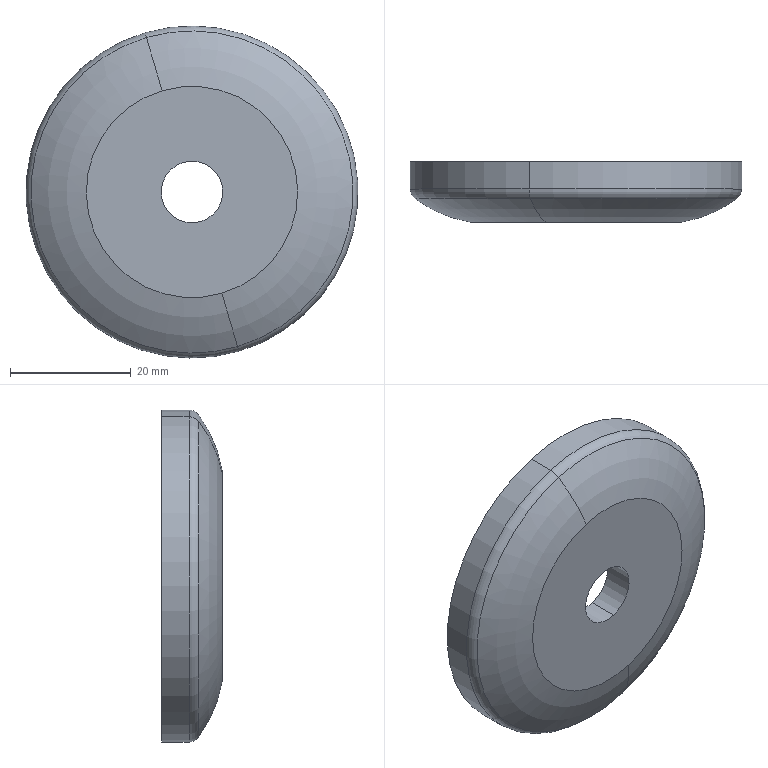Component | SolidWorks | Blade cover-1 | 1 solid | 19 faces | box 55 x 10 x 55 mm | volume 12758 mm3 | cylinder 10 | plane 5 | torus 4 | commonest cylinder face diameters 55 x2 10.2 x2 30 x2 36 x2 49 x2
build123d program:
from build123d import *

# Parameters (mm, degrees)
CONG_1_R = 2


with BuildPart() as part:
    # Esquisse1 → R_volution1 (revolve)
    with BuildSketch(Plane.XY, mode=Mode.PRIVATE) as r_volution1_sk:
        with BuildLine():
            Line((27.5, 0), (27.5, 5.5))
            ThreePointArc((27.5, 5.5), (22.785, 8.383), (17.5, 10))
            Line((17.5, 10), (5.1, 10))
            Line((5.1, 10), (5.1, 5))
            Line((5.1, 5), (15, 5))
            Line((15, 5), (15, 0))
            Line((15, 0), (18, 0))
            Line((18, 0), (18, 5))
            Line((18, 5), (24.5, 5))
            Line((24.5, 5), (24.5, 0))
            Line((24.5, 0), (27.5, 0))
        make_face()
    revolve(r_volution1_sk.sketch.rotate(Axis((0, 0, 0), (0, 1, 0)), 90), axis=Axis((0, 0, 0), (0, 1, 0)))

    # Cong_1
    cong_1_edges = [part.edges().sort_by_distance(p)[0] for p in [
        (0, 5.5, 27.5),
    ]]
    fillet(cong_1_edges, radius=CONG_1_R)


solid = part.part

# Placed as in the assembly
solid = solid.moved(Location((-11.038, -39.3, -47.854), (180, 0, 0)))
STEP:
#1=COLOUR_RGB('',0.7922,0.8196,0.9333);
#2=FILL_AREA_STYLE_COLOUR('',#1);
#3=FILL_AREA_STYLE('',(#2));
#4=SURFACE_STYLE_FILL_AREA(#3);
#5=SURFACE_SIDE_STYLE('',(#4));
#6=SURFACE_STYLE_USAGE(.BOTH.,#5);
#7=PRESENTATION_STYLE_ASSIGNMENT((#6));
#8=CARTESIAN_POINT('',(-0.7406,-1.725,-0.8455));
#9=VERTEX_POINT('',#8);
#10=CARTESIAN_POINT('',(-0.1285,-1.725,-2.923));
#11=VERTEX_POINT('',#10);
#12=CARTESIAN_POINT('',(-0.4346,-1.725,-1.884));
#13=DIRECTION('',(0.,1.,-0.));
#14=DIRECTION('',(0.2827,-0.,-0.9592));
#15=AXIS2_PLACEMENT_3D('',#12,#13,#14);
#16=CIRCLE('',#15,1.083);
#17=EDGE_CURVE('',#9,#11,#16,.T.);
#18=ORIENTED_EDGE('',*,*,#17,.F.);
#19=CARTESIAN_POINT('',(-0.7314,-1.789,-0.8767));
#20=VERTEX_POINT('',#19);
#21=CARTESIAN_POINT('',(-0.7184,-1.725,-0.921));
#22=DIRECTION('',(0.9592,-0.,0.2827));
#23=DIRECTION('',(0.2827,0.,-0.9592));
#24=AXIS2_PLACEMENT_3D('',#21,#22,#23);
#25=CIRCLE('',#24,0.07874);
#26=EDGE_CURVE('',#9,#20,#25,.T.);
#27=ORIENTED_EDGE('',*,*,#26,.T.);
#28=CARTESIAN_POINT('',(-0.1377,-1.789,-2.891));
#29=VERTEX_POINT('',#28);
#30=CARTESIAN_POINT('',(-0.4346,-1.789,-1.884));
#31=DIRECTION('',(-0.,-1.,0.));
#32=DIRECTION('',(-0.2827,0.,0.9592));
#33=AXIS2_PLACEMENT_3D('',#30,#31,#32);
#34=CIRCLE('',#33,1.05);
#35=EDGE_CURVE('',#29,#20,#34,.T.);
#36=ORIENTED_EDGE('',*,*,#35,.F.);
#37=CARTESIAN_POINT('',(-0.1508,-1.725,-2.847));
#38=DIRECTION('',(-0.9592,0.,-0.2827));
#39=DIRECTION('',(-0.2827,0.,0.9592));
#40=AXIS2_PLACEMENT_3D('',#37,#38,#39);
#41=CIRCLE('',#40,0.07874);
#42=EDGE_CURVE('',#11,#29,#41,.T.);
#43=ORIENTED_EDGE('',*,*,#42,.F.);
#44=EDGE_LOOP('',(#18,#27,#36,#43));
#45=FACE_OUTER_BOUND('',#44,.T.);
#46=CARTESIAN_POINT('',(-0.4346,-1.725,-1.884));
#47=DIRECTION('',(-0.,-1.,0.));
#48=DIRECTION('',(0.2827,-0.,-0.9592));
#49=AXIS2_PLACEMENT_3D('',#46,#47,#48);
#50=TOROIDAL_SURFACE('',#49,1.004,0.07874);
#51=ADVANCED_FACE('',(#45),#50,.T.);
#52=ORIENTED_EDGE('',*,*,#17,.T.);
#53=CARTESIAN_POINT('',(-0.1285,-1.547,-2.923));
#54=VERTEX_POINT('',#53);
#55=CARTESIAN_POINT('',(-0.1285,-1.547,-2.923));
#56=DIRECTION('',(0.,1.,-0.));
#57=VECTOR('',#56,39.37);
#58=LINE('',#55,#57);
#59=EDGE_CURVE('',#11,#54,#58,.T.);
#60=ORIENTED_EDGE('',*,*,#59,.T.);
#61=CARTESIAN_POINT('',(-0.7406,-1.547,-0.8455));
#62=VERTEX_POINT('',#61);
#63=CARTESIAN_POINT('',(-0.4346,-1.547,-1.884));
#64=DIRECTION('',(0.,1.,-0.));
#65=DIRECTION('',(-0.2827,0.,0.9592));
#66=AXIS2_PLACEMENT_3D('',#63,#64,#65);
#67=CIRCLE('',#66,1.083);
#68=EDGE_CURVE('',#62,#54,#67,.T.);
#69=ORIENTED_EDGE('',*,*,#68,.F.);
#70=CARTESIAN_POINT('',(-0.7406,-1.547,-0.8455));
#71=DIRECTION('',(0.,1.,-0.));
#72=VECTOR('',#71,39.37);
#73=LINE('',#70,#72);
#74=EDGE_CURVE('',#9,#62,#73,.T.);
#75=ORIENTED_EDGE('',*,*,#74,.F.);
#76=EDGE_LOOP('',(#52,#60,#69,#75));
#77=FACE_OUTER_BOUND('',#76,.T.);
#78=CARTESIAN_POINT('',(-0.4346,-1.547,-1.884));
#79=DIRECTION('',(0.,1.,-0.));
#80=DIRECTION('',(-0.2827,0.,0.9592));
#81=AXIS2_PLACEMENT_3D('',#78,#79,#80);
#82=CYLINDRICAL_SURFACE('',#81,1.083);
#83=ADVANCED_FACE('',(#77),#82,.T.);
#84=CARTESIAN_POINT('',(-0.6293,-1.941,-1.223));
#85=VERTEX_POINT('',#84);
#86=CARTESIAN_POINT('',(-0.2398,-1.941,-2.545));
#87=VERTEX_POINT('',#86);
#88=CARTESIAN_POINT('',(-0.4346,-1.941,-1.884));
#89=DIRECTION('',(0.,1.,-0.));
#90=DIRECTION('',(-0.2827,0.,0.9592));
#91=AXIS2_PLACEMENT_3D('',#88,#89,#90);
#92=CIRCLE('',#91,0.689);
#93=EDGE_CURVE('',#85,#87,#92,.T.);
#94=ORIENTED_EDGE('',*,*,#93,.T.);
#95=CARTESIAN_POINT('',(-0.2815,-1.087,-2.404));
#96=DIRECTION('',(0.9592,-0.,0.2827));
#97=DIRECTION('',(0.2827,0.,-0.9592));
#98=AXIS2_PLACEMENT_3D('',#95,#96,#97);
#99=CIRCLE('',#98,0.8661);
#100=EDGE_CURVE('',#87,#29,#99,.T.);
#101=ORIENTED_EDGE('',*,*,#100,.T.);
#102=ORIENTED_EDGE('',*,*,#35,.T.);
#103=CARTESIAN_POINT('',(-0.5877,-1.087,-1.365));
#104=DIRECTION('',(-0.9592,0.,-0.2827));
#105=DIRECTION('',(-0.2827,0.,0.9592));
#106=AXIS2_PLACEMENT_3D('',#103,#104,#105);
#107=CIRCLE('',#106,0.8661);
#108=EDGE_CURVE('',#85,#20,#107,.T.);
#109=ORIENTED_EDGE('',*,*,#108,.F.);
#110=EDGE_LOOP('',(#94,#101,#102,#109));
#111=FACE_OUTER_BOUND('',#110,.T.);
#112=CARTESIAN_POINT('',(-0.4346,-1.087,-1.884));
#113=DIRECTION('',(0.,1.,-0.));
#114=DIRECTION('',(-0.2827,0.,0.9592));
#115=AXIS2_PLACEMENT_3D('',#112,#113,#114);
#116=TOROIDAL_SURFACE('',#115,0.5416,0.8661);
#117=ADVANCED_FACE('',(#111),#116,.T.);
#118=CARTESIAN_POINT('',(-0.3778,-1.941,-2.077));
#119=VERTEX_POINT('',#118);
#120=CARTESIAN_POINT('',(-0.4913,-1.941,-1.691));
#121=VERTEX_POINT('',#120);
#122=CARTESIAN_POINT('',(-0.4346,-1.941,-1.884));
#123=DIRECTION('',(0.,1.,-0.));
#124=DIRECTION('',(-0.2827,0.,0.9592));
#125=AXIS2_PLACEMENT_3D('',#122,#123,#124);
#126=CIRCLE('',#125,0.2008);
#127=EDGE_CURVE('',#119,#121,#126,.T.);
#128=ORIENTED_EDGE('',*,*,#127,.F.);
#129=CARTESIAN_POINT('',(-0.3778,-1.744,-2.077));
#130=VERTEX_POINT('',#129);
#131=CARTESIAN_POINT('',(-0.3778,-1.547,-2.077));
#132=DIRECTION('',(0.,1.,-0.));
#133=VECTOR('',#132,39.37);
#134=LINE('',#131,#133);
#135=EDGE_CURVE('',#119,#130,#134,.T.);
#136=ORIENTED_EDGE('',*,*,#135,.T.);
#137=CARTESIAN_POINT('',(-0.4913,-1.744,-1.691));
#138=VERTEX_POINT('',#137);
#139=CARTESIAN_POINT('',(-0.4346,-1.744,-1.884));
#140=DIRECTION('',(0.,1.,-0.));
#141=DIRECTION('',(-0.2827,0.,0.9592));
#142=AXIS2_PLACEMENT_3D('',#139,#140,#141);
#143=CIRCLE('',#142,0.2008);
#144=EDGE_CURVE('',#130,#138,#143,.T.);
#145=ORIENTED_EDGE('',*,*,#144,.T.);
#146=CARTESIAN_POINT('',(-0.4913,-1.547,-1.691));
#147=DIRECTION('',(0.,1.,-0.));
#148=VECTOR('',#147,39.37);
#149=LINE('',#146,#148);
#150=EDGE_CURVE('',#121,#138,#149,.T.);
#151=ORIENTED_EDGE('',*,*,#150,.F.);
#152=EDGE_LOOP('',(#128,#136,#145,#151));
#153=FACE_OUTER_BOUND('',#152,.T.);
#154=CARTESIAN_POINT('',(-0.4346,-1.547,-1.884));
#155=DIRECTION('',(0.,1.,-0.));
#156=DIRECTION('',(-0.2827,0.,0.9592));
#157=AXIS2_PLACEMENT_3D('',#154,#155,#156);
#158=CYLINDRICAL_SURFACE('',#157,0.2008);
#159=ADVANCED_FACE('',(#153),#158,.F.);
#160=CARTESIAN_POINT('',(-0.2676,-1.744,-2.45));
#161=VERTEX_POINT('',#160);
#162=CARTESIAN_POINT('',(-0.6015,-1.744,-1.318));
#163=VERTEX_POINT('',#162);
#164=CARTESIAN_POINT('',(-0.4346,-1.744,-1.884));
#165=DIRECTION('',(0.,1.,-0.));
#166=DIRECTION('',(-0.2827,0.,0.9592));
#167=AXIS2_PLACEMENT_3D('',#164,#165,#166);
#168=CIRCLE('',#167,0.5906);
#169=EDGE_CURVE('',#161,#163,#168,.T.);
#170=ORIENTED_EDGE('',*,*,#169,.F.);
#171=CARTESIAN_POINT('',(-0.2676,-1.547,-2.45));
#172=VERTEX_POINT('',#171);
#173=CARTESIAN_POINT('',(-0.2676,-1.547,-2.45));
#174=DIRECTION('',(0.,1.,-0.));
#175=VECTOR('',#174,39.37);
#176=LINE('',#173,#175);
#177=EDGE_CURVE('',#161,#172,#176,.T.);
#178=ORIENTED_EDGE('',*,*,#177,.T.);
#179=CARTESIAN_POINT('',(-0.6015,-1.547,-1.318));
#180=VERTEX_POINT('',#179);
#181=CARTESIAN_POINT('',(-0.4346,-1.547,-1.884));
#182=DIRECTION('',(0.,1.,-0.));
#183=DIRECTION('',(-0.2827,0.,0.9592));
#184=AXIS2_PLACEMENT_3D('',#181,#182,#183);
#185=CIRCLE('',#184,0.5906);
#186=EDGE_CURVE('',#172,#180,#185,.T.);
#187=ORIENTED_EDGE('',*,*,#186,.T.);
#188=CARTESIAN_POINT('',(-0.6015,-1.547,-1.318));
#189=DIRECTION('',(0.,1.,-0.));
#190=VECTOR('',#189,39.37);
#191=LINE('',#188,#190);
#192=EDGE_CURVE('',#163,#180,#191,.T.);
#193=ORIENTED_EDGE('',*,*,#192,.F.);
#194=EDGE_LOOP('',(#170,#178,#187,#193));
#195=FACE_OUTER_BOUND('',#194,.T.);
#196=CARTESIAN_POINT('',(-0.4346,-1.547,-1.884));
#197=DIRECTION('',(0.,1.,-0.));
#198=DIRECTION('',(-0.2827,0.,0.9592));
#199=AXIS2_PLACEMENT_3D('',#196,#197,#198);
#200=CYLINDRICAL_SURFACE('',#199,0.5906);
#201=ADVANCED_FACE('',(#195),#200,.F.);
#202=CARTESIAN_POINT('',(-0.6349,-1.744,-1.204));
#203=VERTEX_POINT('',#202);
#204=CARTESIAN_POINT('',(-0.2343,-1.744,-2.564));
#205=VERTEX_POINT('',#204);
#206=CARTESIAN_POINT('',(-0.4346,-1.744,-1.884));
#207=DIRECTION('',(0.,1.,-0.));
#208=DIRECTION('',(-0.2827,0.,0.9592));
#209=AXIS2_PLACEMENT_3D('',#206,#207,#208);
#210=CIRCLE('',#209,0.7087);
#211=EDGE_CURVE('',#203,#205,#210,.T.);
#212=ORIENTED_EDGE('',*,*,#211,.T.);
#213=CARTESIAN_POINT('',(-0.2343,-1.547,-2.564));
#214=VERTEX_POINT('',#213);
#215=CARTESIAN_POINT('',(-0.2343,-1.547,-2.564));
#216=DIRECTION('',(0.,1.,-0.));
#217=VECTOR('',#216,39.37);
#218=LINE('',#215,#217);
#219=EDGE_CURVE('',#205,#214,#218,.T.);
#220=ORIENTED_EDGE('',*,*,#219,.T.);
#221=CARTESIAN_POINT('',(-0.6349,-1.547,-1.204));
#222=VERTEX_POINT('',#221);
#223=CARTESIAN_POINT('',(-0.4346,-1.547,-1.884));
#224=DIRECTION('',(0.,1.,-0.));
#225=DIRECTION('',(-0.2827,0.,0.9592));
#226=AXIS2_PLACEMENT_3D('',#223,#224,#225);
#227=CIRCLE('',#226,0.7087);
#228=EDGE_CURVE('',#222,#214,#227,.T.);
#229=ORIENTED_EDGE('',*,*,#228,.F.);
#230=CARTESIAN_POINT('',(-0.6349,-1.547,-1.204));
#231=DIRECTION('',(0.,1.,-0.));
#232=VECTOR('',#231,39.37);
#233=LINE('',#230,#232);
#234=EDGE_CURVE('',#203,#222,#233,.T.);
#235=ORIENTED_EDGE('',*,*,#234,.F.);
#236=EDGE_LOOP('',(#212,#220,#229,#235));
#237=FACE_OUTER_BOUND('',#236,.T.);
#238=CARTESIAN_POINT('',(-0.4346,-1.547,-1.884));
#239=DIRECTION('',(0.,1.,-0.));
#240=DIRECTION('',(-0.2827,0.,0.9592));
#241=AXIS2_PLACEMENT_3D('',#238,#239,#240);
#242=CYLINDRICAL_SURFACE('',#241,0.7087);
#243=ADVANCED_FACE('',(#237),#242,.T.);
#244=CARTESIAN_POINT('',(-0.1619,-1.744,-2.809));
#245=VERTEX_POINT('',#244);
#246=CARTESIAN_POINT('',(-0.7072,-1.744,-0.9588));
#247=VERTEX_POINT('',#246);
#248=CARTESIAN_POINT('',(-0.4346,-1.744,-1.884));
#249=DIRECTION('',(0.,1.,-0.));
#250=DIRECTION('',(-0.2827,0.,0.9592));
#251=AXIS2_PLACEMENT_3D('',#248,#249,#250);
#252=CIRCLE('',#251,0.9646);
#253=EDGE_CURVE('',#245,#247,#252,.T.);
#254=ORIENTED_EDGE('',*,*,#253,.F.);
#255=CARTESIAN_POINT('',(-0.1619,-1.547,-2.809));
#256=VERTEX_POINT('',#255);
#257=CARTESIAN_POINT('',(-0.1619,-1.547,-2.809));
#258=DIRECTION('',(0.,1.,-0.));
#259=VECTOR('',#258,39.37);
#260=LINE('',#257,#259);
#261=EDGE_CURVE('',#245,#256,#260,.T.);
#262=ORIENTED_EDGE('',*,*,#261,.T.);
#263=CARTESIAN_POINT('',(-0.7072,-1.547,-0.9588));
#264=VERTEX_POINT('',#263);
#265=CARTESIAN_POINT('',(-0.4346,-1.547,-1.884));
#266=DIRECTION('',(0.,1.,-0.));
#267=DIRECTION('',(-0.2827,0.,0.9592));
#268=AXIS2_PLACEMENT_3D('',#265,#266,#267);
#269=CIRCLE('',#268,0.9646);
#270=EDGE_CURVE('',#256,#264,#269,.T.);
#271=ORIENTED_EDGE('',*,*,#270,.T.);
#272=CARTESIAN_POINT('',(-0.7072,-1.547,-0.9588));
#273=DIRECTION('',(0.,1.,-0.));
#274=VECTOR('',#273,39.37);
#275=LINE('',#272,#274);
#276=EDGE_CURVE('',#247,#264,#275,.T.);
#277=ORIENTED_EDGE('',*,*,#276,.F.);
#278=EDGE_LOOP('',(#254,#262,#271,#277));
#279=FACE_OUTER_BOUND('',#278,.T.);
#280=CARTESIAN_POINT('',(-0.4346,-1.547,-1.884));
#281=DIRECTION('',(0.,1.,-0.));
#282=DIRECTION('',(-0.2827,0.,0.9592));
#283=AXIS2_PLACEMENT_3D('',#280,#281,#282);
#284=CYLINDRICAL_SURFACE('',#283,0.9646);
#285=ADVANCED_FACE('',(#279),#284,.F.);
#286=ORIENTED_EDGE('',*,*,#68,.T.);
#287=CARTESIAN_POINT('',(-0.4346,-1.547,-1.884));
#288=DIRECTION('',(0.,1.,-0.));
#289=DIRECTION('',(-0.2827,0.,0.9592));
#290=AXIS2_PLACEMENT_3D('',#287,#288,#289);
#291=CIRCLE('',#290,1.083);
#292=EDGE_CURVE('',#54,#62,#291,.T.);
#293=ORIENTED_EDGE('',*,*,#292,.T.);
#294=EDGE_LOOP('',(#286,#293));
#295=FACE_OUTER_BOUND('',#294,.T.);
#296=CARTESIAN_POINT('',(-0.4346,-1.547,-1.884));
#297=DIRECTION('',(0.,1.,-0.));
#298=DIRECTION('',(-0.2827,0.,0.9592));
#299=AXIS2_PLACEMENT_3D('',#296,#297,#298);
#300=CIRCLE('',#299,0.9646);
#301=EDGE_CURVE('',#264,#256,#300,.T.);
#302=ORIENTED_EDGE('',*,*,#301,.F.);
#303=ORIENTED_EDGE('',*,*,#270,.F.);
#304=EDGE_LOOP('',(#302,#303));
#305=FACE_BOUND('',#304,.T.);
#306=CARTESIAN_POINT('',(0.4906,-1.547,-1.611));
#307=DIRECTION('',(0.,1.,-0.));
#308=DIRECTION('',(-0.2827,0.,0.9592));
#309=AXIS2_PLACEMENT_3D('',#306,#307,#308);
#310=PLANE('',#309);
#311=ADVANCED_FACE('',(#295,#305),#310,.T.);
#312=ORIENTED_EDGE('',*,*,#261,.F.);
#313=CARTESIAN_POINT('',(-0.4346,-1.744,-1.884));
#314=DIRECTION('',(0.,1.,-0.));
#315=DIRECTION('',(-0.2827,0.,0.9592));
#316=AXIS2_PLACEMENT_3D('',#313,#314,#315);
#317=CIRCLE('',#316,0.9646);
#318=EDGE_CURVE('',#247,#245,#317,.T.);
#319=ORIENTED_EDGE('',*,*,#318,.F.);
#320=ORIENTED_EDGE('',*,*,#276,.T.);
#321=ORIENTED_EDGE('',*,*,#301,.T.);
#322=EDGE_LOOP('',(#312,#319,#320,#321));
#323=FACE_OUTER_BOUND('',#322,.T.);
#324=CARTESIAN_POINT('',(-0.4346,-1.547,-1.884));
#325=DIRECTION('',(0.,1.,-0.));
#326=DIRECTION('',(-0.2827,0.,0.9592));
#327=AXIS2_PLACEMENT_3D('',#324,#325,#326);
#328=CYLINDRICAL_SURFACE('',#327,0.9646);
#329=ADVANCED_FACE('',(#323),#328,.F.);
#330=ORIENTED_EDGE('',*,*,#318,.T.);
#331=ORIENTED_EDGE('',*,*,#253,.T.);
#332=EDGE_LOOP('',(#330,#331));
#333=FACE_OUTER_BOUND('',#332,.T.);
#334=ORIENTED_EDGE('',*,*,#211,.F.);
#335=CARTESIAN_POINT('',(-0.4346,-1.744,-1.884));
#336=DIRECTION('',(0.,1.,-0.));
#337=DIRECTION('',(-0.2827,0.,0.9592));
#338=AXIS2_PLACEMENT_3D('',#335,#336,#337);
#339=CIRCLE('',#338,0.7087);
#340=EDGE_CURVE('',#205,#203,#339,.T.);
#341=ORIENTED_EDGE('',*,*,#340,.F.);
#342=EDGE_LOOP('',(#334,#341));
#343=FACE_BOUND('',#342,.T.);
#344=CARTESIAN_POINT('',(0.2452,-1.744,-1.684));
#345=DIRECTION('',(0.,1.,-0.));
#346=DIRECTION('',(-0.2827,0.,0.9592));
#347=AXIS2_PLACEMENT_3D('',#344,#345,#346);
#348=PLANE('',#347);
#349=ADVANCED_FACE('',(#333,#343),#348,.T.);
#350=ORIENTED_EDGE('',*,*,#219,.F.);
#351=ORIENTED_EDGE('',*,*,#340,.T.);
#352=ORIENTED_EDGE('',*,*,#234,.T.);
#353=CARTESIAN_POINT('',(-0.4346,-1.547,-1.884));
#354=DIRECTION('',(0.,1.,-0.));
#355=DIRECTION('',(-0.2827,0.,0.9592));
#356=AXIS2_PLACEMENT_3D('',#353,#354,#355);
#357=CIRCLE('',#356,0.7087);
#358=EDGE_CURVE('',#214,#222,#357,.T.);
#359=ORIENTED_EDGE('',*,*,#358,.F.);
#360=EDGE_LOOP('',(#350,#351,#352,#359));
#361=FACE_OUTER_BOUND('',#360,.T.);
#362=CARTESIAN_POINT('',(-0.4346,-1.547,-1.884));
#363=DIRECTION('',(0.,1.,-0.));
#364=DIRECTION('',(-0.2827,0.,0.9592));
#365=AXIS2_PLACEMENT_3D('',#362,#363,#364);
#366=CYLINDRICAL_SURFACE('',#365,0.7087);
#367=ADVANCED_FACE('',(#361),#366,.T.);
#368=ORIENTED_EDGE('',*,*,#228,.T.);
#369=ORIENTED_EDGE('',*,*,#358,.T.);
#370=EDGE_LOOP('',(#368,#369));
#371=FACE_OUTER_BOUND('',#370,.T.);
#372=CARTESIAN_POINT('',(-0.4346,-1.547,-1.884));
#373=DIRECTION('',(0.,1.,-0.));
#374=DIRECTION('',(-0.2827,0.,0.9592));
#375=AXIS2_PLACEMENT_3D('',#372,#373,#374);
#376=CIRCLE('',#375,0.5906);
#377=EDGE_CURVE('',#180,#172,#376,.T.);
#378=ORIENTED_EDGE('',*,*,#377,.F.);
#379=ORIENTED_EDGE('',*,*,#186,.F.);
#380=EDGE_LOOP('',(#378,#379));
#381=FACE_BOUND('',#380,.T.);
#382=CARTESIAN_POINT('',(0.1319,-1.547,-1.717));
#383=DIRECTION('',(0.,1.,-0.));
#384=DIRECTION('',(-0.2827,0.,0.9592));
#385=AXIS2_PLACEMENT_3D('',#382,#383,#384);
#386=PLANE('',#385);
#387=ADVANCED_FACE('',(#371,#381),#386,.T.);
#388=ORIENTED_EDGE('',*,*,#177,.F.);
#389=CARTESIAN_POINT('',(-0.4346,-1.744,-1.884));
#390=DIRECTION('',(0.,1.,-0.));
#391=DIRECTION('',(-0.2827,0.,0.9592));
#392=AXIS2_PLACEMENT_3D('',#389,#390,#391);
#393=CIRCLE('',#392,0.5906);
#394=EDGE_CURVE('',#163,#161,#393,.T.);
#395=ORIENTED_EDGE('',*,*,#394,.F.);
#396=ORIENTED_EDGE('',*,*,#192,.T.);
#397=ORIENTED_EDGE('',*,*,#377,.T.);
#398=EDGE_LOOP('',(#388,#395,#396,#397));
#399=FACE_OUTER_BOUND('',#398,.T.);
#400=CARTESIAN_POINT('',(-0.4346,-1.547,-1.884));
#401=DIRECTION('',(0.,1.,-0.));
#402=DIRECTION('',(-0.2827,0.,0.9592));
#403=AXIS2_PLACEMENT_3D('',#400,#401,#402);
#404=CYLINDRICAL_SURFACE('',#403,0.5906);
#405=ADVANCED_FACE('',(#399),#404,.F.);
#406=ORIENTED_EDGE('',*,*,#394,.T.);
#407=ORIENTED_EDGE('',*,*,#169,.T.);
#408=EDGE_LOOP('',(#406,#407));
#409=FACE_OUTER_BOUND('',#408,.T.);
#410=CARTESIAN_POINT('',(-0.4346,-1.744,-1.884));
#411=DIRECTION('',(0.,1.,-0.));
#412=DIRECTION('',(-0.2827,0.,0.9592));
#413=AXIS2_PLACEMENT_3D('',#410,#411,#412);
#414=CIRCLE('',#413,0.2008);
#415=EDGE_CURVE('',#138,#130,#414,.T.);
#416=ORIENTED_EDGE('',*,*,#415,.F.);
#417=ORIENTED_EDGE('',*,*,#144,.F.);
#418=EDGE_LOOP('',(#416,#417));
#419=FACE_BOUND('',#418,.T.);
#420=CARTESIAN_POINT('',(-0.242,-1.744,-1.827));
#421=DIRECTION('',(0.,1.,-0.));
#422=DIRECTION('',(-0.2827,0.,0.9592));
#423=AXIS2_PLACEMENT_3D('',#420,#421,#422);
#424=PLANE('',#423);
#425=ADVANCED_FACE('',(#409,#419),#424,.T.);
#426=ORIENTED_EDGE('',*,*,#135,.F.);
#427=CARTESIAN_POINT('',(-0.4346,-1.941,-1.884));
#428=DIRECTION('',(0.,1.,-0.));
#429=DIRECTION('',(-0.2827,0.,0.9592));
#430=AXIS2_PLACEMENT_3D('',#427,#428,#429);
#431=CIRCLE('',#430,0.2008);
#432=EDGE_CURVE('',#121,#119,#431,.T.);
#433=ORIENTED_EDGE('',*,*,#432,.F.);
#434=ORIENTED_EDGE('',*,*,#150,.T.);
#435=ORIENTED_EDGE('',*,*,#415,.T.);
#436=EDGE_LOOP('',(#426,#433,#434,#435));
#437=FACE_OUTER_BOUND('',#436,.T.);
#438=CARTESIAN_POINT('',(-0.4346,-1.547,-1.884));
#439=DIRECTION('',(0.,1.,-0.));
#440=DIRECTION('',(-0.2827,0.,0.9592));
#441=AXIS2_PLACEMENT_3D('',#438,#439,#440);
#442=CYLINDRICAL_SURFACE('',#441,0.2008);
#443=ADVANCED_FACE('',(#437),#442,.F.);
#444=ORIENTED_EDGE('',*,*,#432,.T.);
#445=ORIENTED_EDGE('',*,*,#127,.T.);
#446=EDGE_LOOP('',(#444,#445));
#447=FACE_BOUND('',#446,.T.);
#448=ORIENTED_EDGE('',*,*,#93,.F.);
#449=CARTESIAN_POINT('',(-0.4346,-1.941,-1.884));
#450=DIRECTION('',(0.,1.,-0.));
#451=DIRECTION('',(-0.2827,0.,0.9592));
#452=AXIS2_PLACEMENT_3D('',#449,#450,#451);
#453=CIRCLE('',#452,0.689);
#454=EDGE_CURVE('',#87,#85,#453,.T.);
#455=ORIENTED_EDGE('',*,*,#454,.F.);
#456=EDGE_LOOP('',(#448,#455));
#457=FACE_OUTER_BOUND('',#456,.T.);
#458=CARTESIAN_POINT('',(-0.242,-1.941,-1.827));
#459=DIRECTION('',(-0.,-1.,0.));
#460=DIRECTION('',(0.2827,-0.,-0.9592));
#461=AXIS2_PLACEMENT_3D('',#458,#459,#460);
#462=PLANE('',#461);
#463=ADVANCED_FACE('',(#447,#457),#462,.T.);
#464=ORIENTED_EDGE('',*,*,#100,.F.);
#465=ORIENTED_EDGE('',*,*,#454,.T.);
#466=ORIENTED_EDGE('',*,*,#108,.T.);
#467=CARTESIAN_POINT('',(-0.4346,-1.789,-1.884));
#468=DIRECTION('',(-0.,-1.,0.));
#469=DIRECTION('',(-0.2827,0.,0.9592));
#470=AXIS2_PLACEMENT_3D('',#467,#468,#469);
#471=CIRCLE('',#470,1.05);
#472=EDGE_CURVE('',#20,#29,#471,.T.);
#473=ORIENTED_EDGE('',*,*,#472,.T.);
#474=EDGE_LOOP('',(#464,#465,#466,#473));
#475=FACE_OUTER_BOUND('',#474,.T.);
#476=CARTESIAN_POINT('',(-0.4346,-1.087,-1.884));
#477=DIRECTION('',(0.,1.,-0.));
#478=DIRECTION('',(-0.2827,0.,0.9592));
#479=AXIS2_PLACEMENT_3D('',#476,#477,#478);
#480=TOROIDAL_SURFACE('',#479,0.5416,0.8661);
#481=ADVANCED_FACE('',(#475),#480,.T.);
#482=ORIENTED_EDGE('',*,*,#59,.F.);
#483=CARTESIAN_POINT('',(-0.4346,-1.725,-1.884));
#484=DIRECTION('',(0.,1.,-0.));
#485=DIRECTION('',(0.2827,-0.,-0.9592));
#486=AXIS2_PLACEMENT_3D('',#483,#484,#485);
#487=CIRCLE('',#486,1.083);
#488=EDGE_CURVE('',#11,#9,#487,.T.);
#489=ORIENTED_EDGE('',*,*,#488,.T.);
#490=ORIENTED_EDGE('',*,*,#74,.T.);
#491=ORIENTED_EDGE('',*,*,#292,.F.);
#492=EDGE_LOOP('',(#482,#489,#490,#491));
#493=FACE_OUTER_BOUND('',#492,.T.);
#494=CARTESIAN_POINT('',(-0.4346,-1.547,-1.884));
#495=DIRECTION('',(0.,1.,-0.));
#496=DIRECTION('',(-0.2827,0.,0.9592));
#497=AXIS2_PLACEMENT_3D('',#494,#495,#496);
#498=CYLINDRICAL_SURFACE('',#497,1.083);
#499=ADVANCED_FACE('',(#493),#498,.T.);
#500=ORIENTED_EDGE('',*,*,#26,.F.);
#501=ORIENTED_EDGE('',*,*,#488,.F.);
#502=ORIENTED_EDGE('',*,*,#42,.T.);
#503=ORIENTED_EDGE('',*,*,#472,.F.);
#504=EDGE_LOOP('',(#500,#501,#502,#503));
#505=FACE_OUTER_BOUND('',#504,.T.);
#506=CARTESIAN_POINT('',(-0.4346,-1.725,-1.884));
#507=DIRECTION('',(-0.,-1.,0.));
#508=DIRECTION('',(0.2827,-0.,-0.9592));
#509=AXIS2_PLACEMENT_3D('',#506,#507,#508);
#510=TOROIDAL_SURFACE('',#509,1.004,0.07874);
#511=ADVANCED_FACE('',(#505),#510,.T.);
#512=CLOSED_SHELL('',(#51,#83,#117,#159,#201,#243,#285,#311,#329,#349,#367,#387,#405,#425,#443,#463,#481,#499,#511));
#513=MANIFOLD_SOLID_BREP('',#512);
#514=STYLED_ITEM('',(#7),#513);
#515=PRESENTATION_LAYER_ASSIGNMENT('','',(#514));
#516=CARTESIAN_POINT('',(0.,0.,0.));
#517=DIRECTION('',(0.,0.,1.));
#518=DIRECTION('',(1.,0.,0.));
#519=AXIS2_PLACEMENT_3D('',#516,#517,#518);
#520=(LENGTH_UNIT()NAMED_UNIT(*)SI_UNIT($,.METRE.));
#521=LENGTH_MEASURE_WITH_UNIT(LENGTH_MEASURE(0.0254),#520);
#522=DIMENSIONAL_EXPONENTS(1.,0.,0.,0.,0.,0.,0.);
#523=(CONVERSION_BASED_UNIT('',#521)LENGTH_UNIT()NAMED_UNIT(#522));
#524=UNCERTAINTY_MEASURE_WITH_UNIT(LENGTH_MEASURE(0.00001),#523,'','');
#525=(NAMED_UNIT(*)PLANE_ANGLE_UNIT()SI_UNIT($,.RADIAN.));
#526=(NAMED_UNIT(*)SI_UNIT($,.STERADIAN.)SOLID_ANGLE_UNIT());
#527=(GEOMETRIC_REPRESENTATION_CONTEXT(3)GLOBAL_UNCERTAINTY_ASSIGNED_CONTEXT((#524))GLOBAL_UNIT_ASSIGNED_CONTEXT((#523,#525,#526))REPRESENTATION_CONTEXT('',''));
#528=ADVANCED_BREP_SHAPE_REPRESENTATION('',(#513,#519),#527);
#529=(LENGTH_UNIT()NAMED_UNIT(*)SI_UNIT($,.METRE.));
#530=LENGTH_MEASURE_WITH_UNIT(LENGTH_MEASURE(0.0254),#529);
#531=DIMENSIONAL_EXPONENTS(1.,0.,0.,0.,0.,0.,0.);
#532=(CONVERSION_BASED_UNIT('',#530)LENGTH_UNIT()NAMED_UNIT(#531));
#533=UNCERTAINTY_MEASURE_WITH_UNIT(LENGTH_MEASURE(0.00001),#532,'','');
#534=(NAMED_UNIT(*)PLANE_ANGLE_UNIT()SI_UNIT($,.RADIAN.));
#535=(NAMED_UNIT(*)SI_UNIT($,.STERADIAN.)SOLID_ANGLE_UNIT());
#536=(GEOMETRIC_REPRESENTATION_CONTEXT(3)GLOBAL_UNCERTAINTY_ASSIGNED_CONTEXT((#533))GLOBAL_UNIT_ASSIGNED_CONTEXT((#532,#534,#535))REPRESENTATION_CONTEXT('',''));
#537=MECHANICAL_DESIGN_GEOMETRIC_PRESENTATION_REPRESENTATION('',(#514),#536);